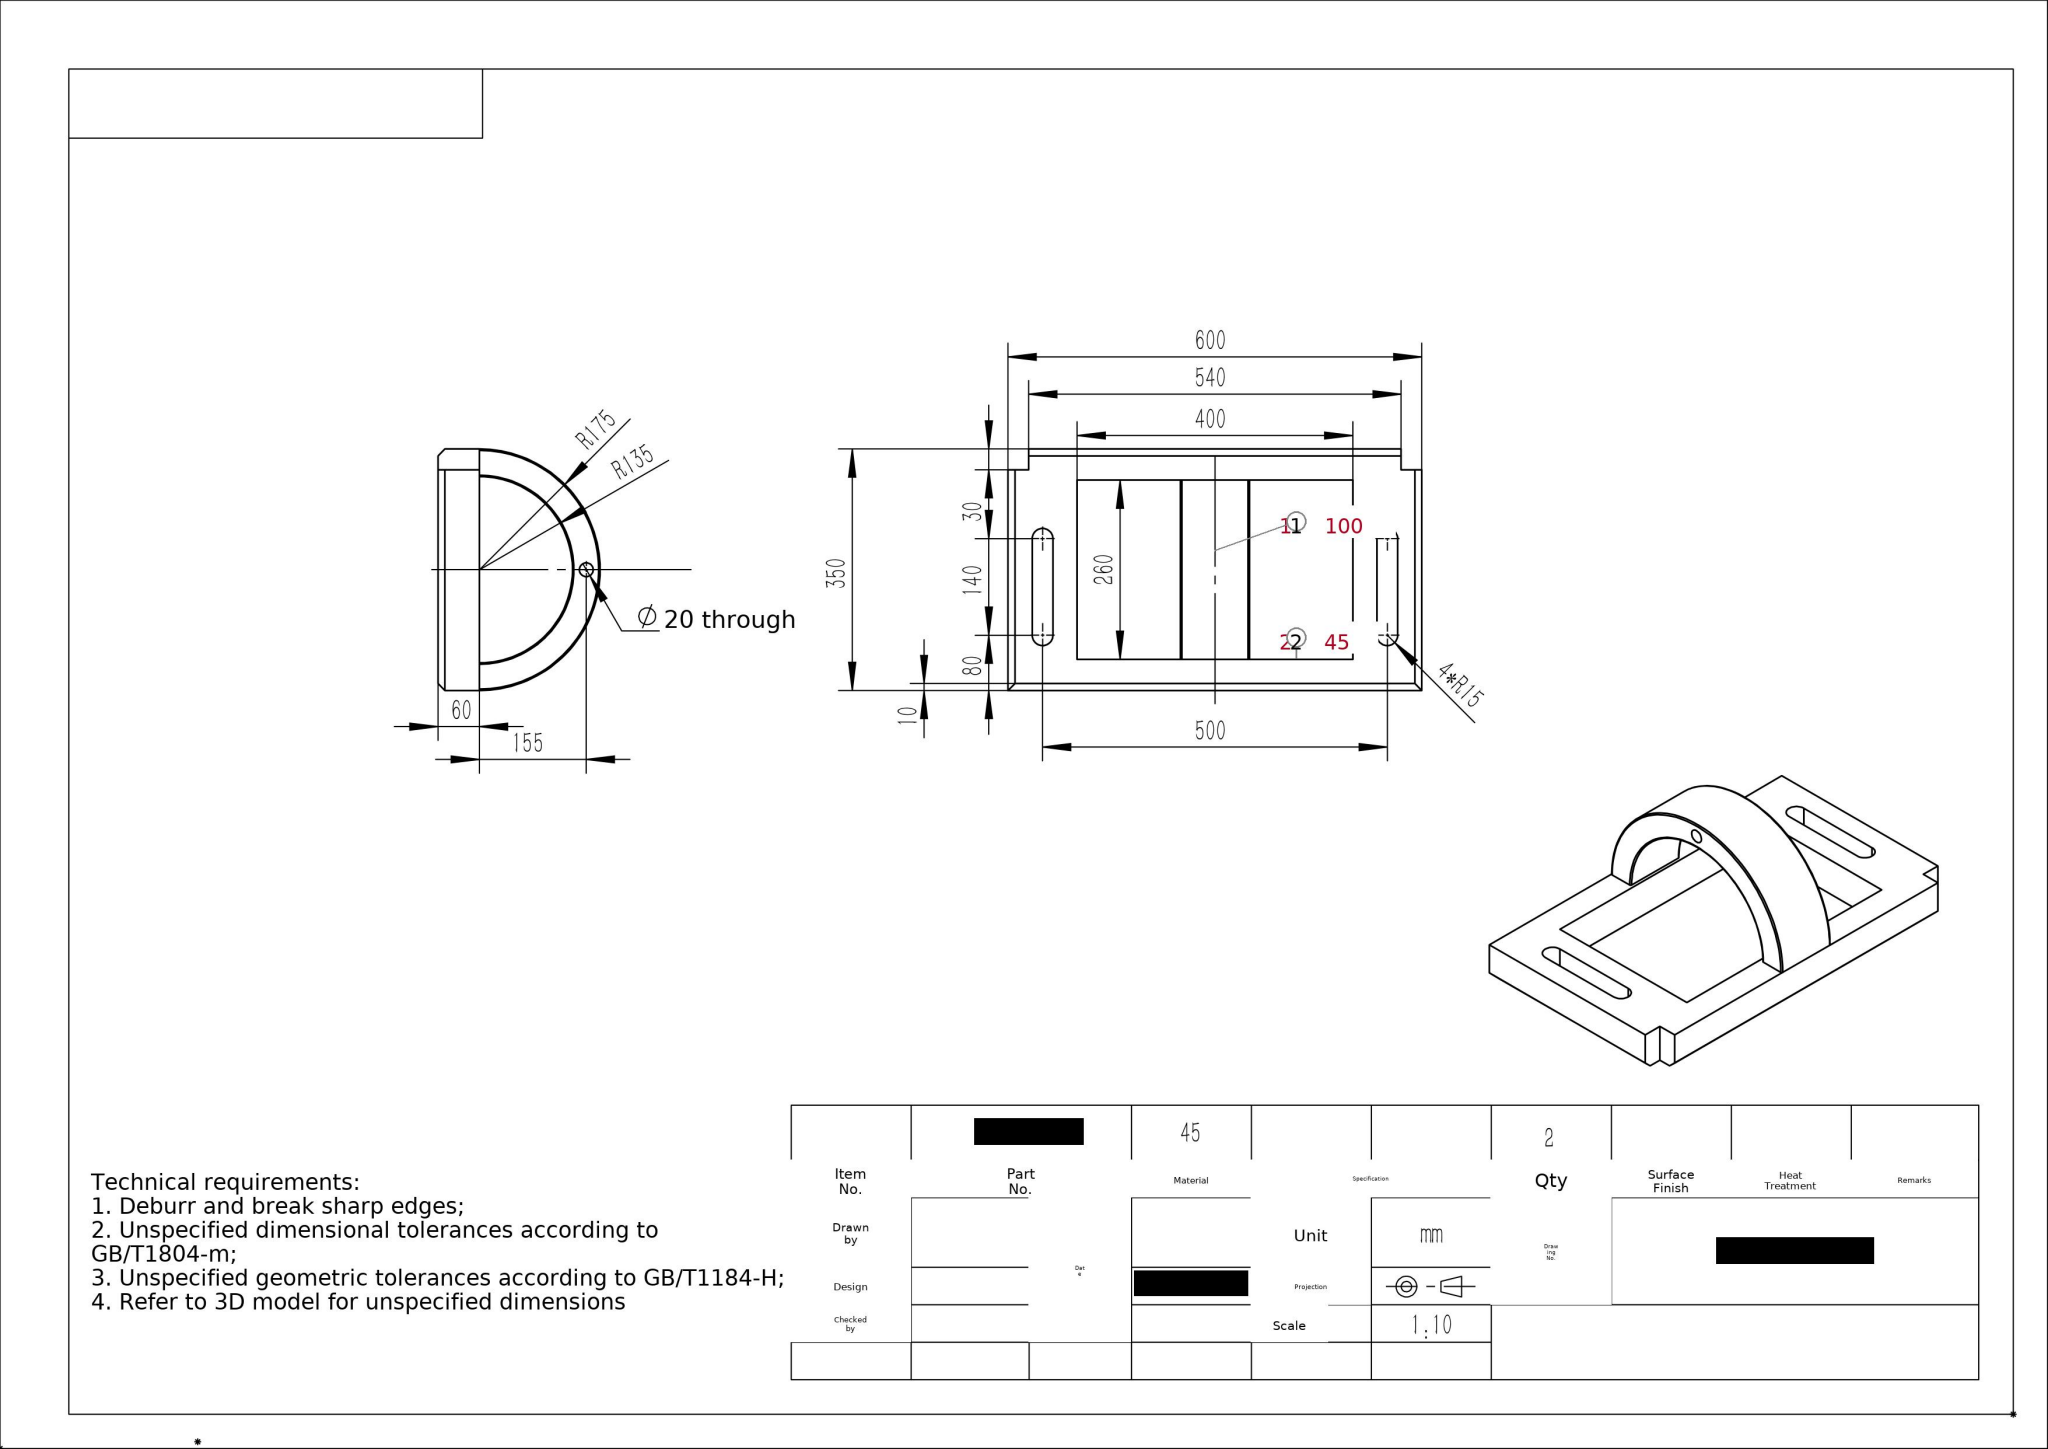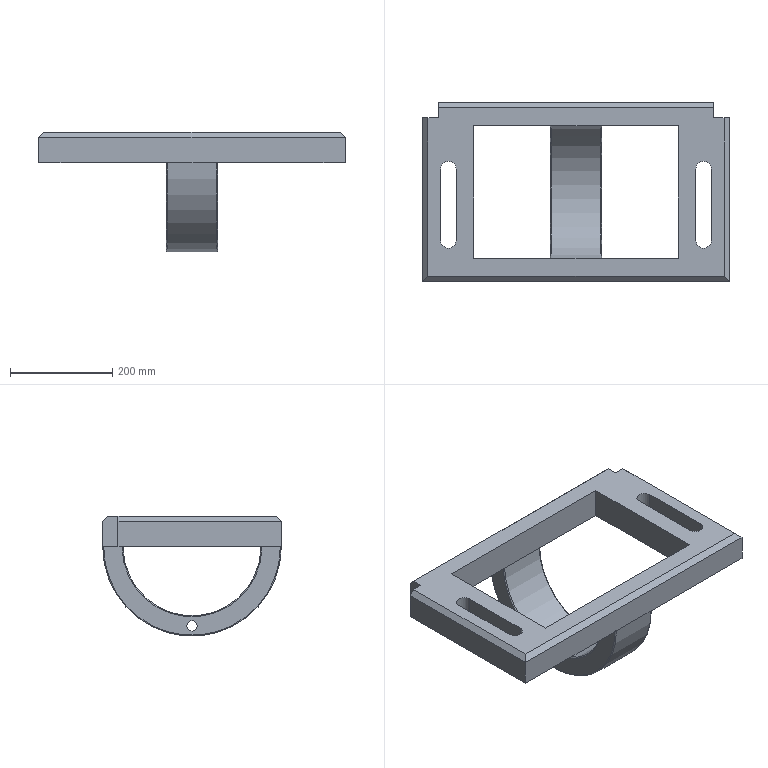Part | SolidWorks | mm | material 45 | 1 solid | 36 faces | box 600 x 350 x 235 mm | volume 7489543 mm3 | plane 24 | cylinder 8 | torus 4 | commonest cylinder face diameters 30 x4 20 x2 350 x1 270 x1
build123d program:
from build123d import *

# Parameters (mm, degrees)
SKETCH1_W           = 600
SKETCH1_H           = 350
SKETCH1_W_2         = 400
SKETCH1_H_2         = 260
BOSS_EXTRUDE1_DEPTH = 60
BOSS_EXTRUDE2_DEPTH = 50
SKETCH3_R           = 10
CUT_EXTRUDE1_DEPTH  = 100
FILLET1_R           = 2
CHAMFER1_SIZE       = 10
SKETCH4_W           = 60
SKETCH4_H           = 60
CUT_EXTRUDE2_DEPTH  = 100


with BuildPart() as part:
    # Sketch1 → Boss-Extrude1 (new body)
    with BuildSketch(Plane.XY):
        Rectangle(SKETCH1_W, SKETCH1_H)
        Rectangle(SKETCH1_W_2, SKETCH1_H_2, mode=Mode.SUBTRACT)
        with BuildLine():
            Line((-235, 45), (-235, -95))
            ThreePointArc((-235, -95), (-250, -110), (-265, -95))
            Line((-265, -95), (-265, 45))
            ThreePointArc((-265, 45), (-250, 60), (-235, 45))
        make_face(mode=Mode.SUBTRACT)
        with BuildLine():
            Line((265, 45), (265, -95))
            ThreePointArc((265, -95), (250, -110), (235, -95))
            Line((235, -95), (235, 45))
            ThreePointArc((235, 45), (250, 60), (265, 45))
        make_face(mode=Mode.SUBTRACT)
    extrude(amount=BOSS_EXTRUDE1_DEPTH)

    # Sketch2 → Boss-Extrude2 (add, symmetric)
    with BuildSketch(Plane(origin=(0, 0, 0), x_dir=(0, 0, -1), z_dir=(1, 0, 0))):
        with BuildLine():
            Line((0, -175), (0, -135))
            ThreePointArc((0, -135), (135, 0), (0, 135))
            Line((0, 135), (0, 175))
            ThreePointArc((0, 175), (175, 0), (0, -175))
        make_face()
    extrude(amount=BOSS_EXTRUDE2_DEPTH, both=True)

    # Sketch3 → Cut-Extrude1 (cut)
    with BuildSketch(Plane(origin=(50, 0, 0), x_dir=(0, 0, -1), z_dir=(1, 0, 0))):
        with Locations((155, 0)):
            Circle(SKETCH3_R)
    extrude(amount=-CUT_EXTRUDE1_DEPTH, mode=Mode.SUBTRACT)

    # Fillet1
    fillet1_edges = [part.edges().sort_by_distance(p)[0] for p in [
        (-50, 0, -175),
        (-50, 0, -135),
        (50, 0, -175),
        (50, 0, -135),
    ]]
    fillet(fillet1_edges, radius=FILLET1_R)

    # Chamfer1
    chamfer1_edges = [part.edges().sort_by_distance(p)[0] for p in [
        (-300, 0, 60),
        (0, -175, 60),
        (300, 0, 60),
        (0, 175, 60),
    ]]
    chamfer(chamfer1_edges, length=CHAMFER1_SIZE)

    # Sketch4 → Cut-Extrude2 (cut)
    with BuildSketch(Plane(origin=(0, 0, 0), x_dir=(-1, 0, 0), z_dir=(0, 0, -1))):
        with Locations((-300, 175)):
            Rectangle(SKETCH4_W, SKETCH4_H)
    cut_extrude2 = extrude(amount=-CUT_EXTRUDE2_DEPTH, mode=Mode.SUBTRACT)

    # Mirror1: Cut-Extrude2 across plane
    add(cut_extrude2.mirror(Plane(origin=(0, 0, 0), x_dir=(0, 0, 1), z_dir=(1, 0, 0))), mode=Mode.SUBTRACT)


solid = part.part